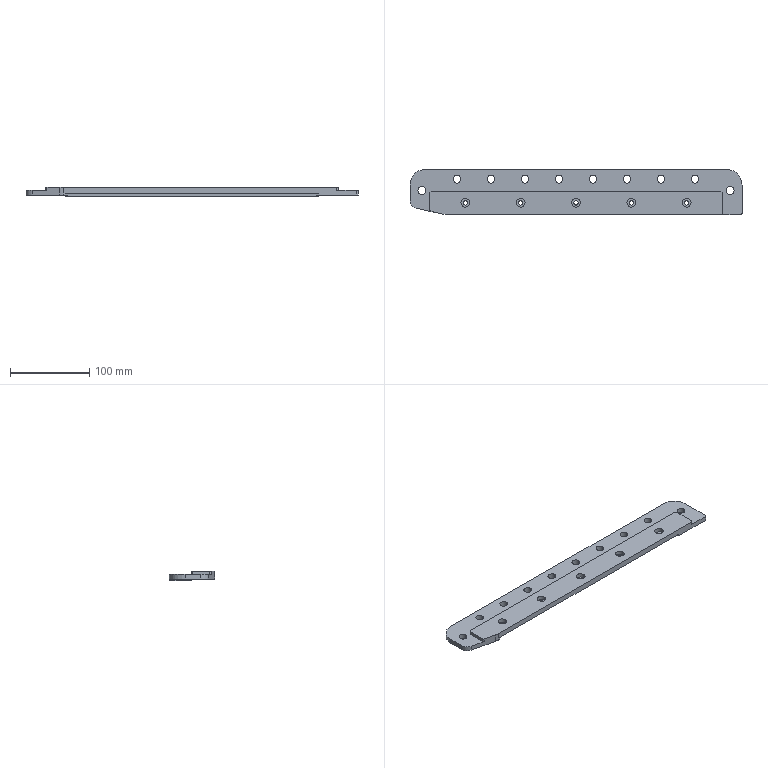Component | SolidWorks | 170423A4-PulleyRetainingPlate2-1 | 1 solid | 80 faces | box 420 x 57.5 x 12 mm | volume 171578 mm3 | cylinder 54 | plane 26 | commonest cylinder face diameters 10 x20 11 x10 5.5 x10 4 x7 2 x3 40 x3 20 x1
build123d program:
from build123d import *

# Parameters (mm, degrees)
SKETCH1_W                                       = 420
SKETCH1_H                                       = 57.5
BOSS_EXTRUDE1_DEPTH                             = 6
F_10_0_10_DIAMETER_HOLE1_D                      = 10
SKETCH4_W                                       = 320.2
SKETCH4_H                                       = 30
CUT_EXTRUDE1_DEPTH                              = 2.5
FILLET1_R                                       = 20
SKETCH9_W                                       = 320.2
SKETCH9_H                                       = 27.5
BOSS_EXTRUDE2_DEPTH                             = 2
F_10_0_10_DIAMETER_HOLE2_D                      = 10
SKETCH10_W                                      = 370
SKETCH10_H                                      = 30
BOSS_EXTRUDE3_DEPTH                             = 4
CHAMFER1_SIZE                                   = 10
CHAMFER1_SIZE2                                  = 45
FILLET2_R                                       = 10
FILLET3_R                                       = 20
FILLET4_R                                       = 2
CUT_EXTRUDE2_DEPTH                              = 2.5
CHAMFER2_SIZE                                   = 2
M5_HEX_SOCKET_HEAD_CAP_SCREW_CBORE1_D           = 5.5
M5_HEX_SOCKET_HEAD_CAP_SCREW_CBORE1_CBORE_D     = 11
M5_HEX_SOCKET_HEAD_CAP_SCREW_CBORE1_CBORE_DEPTH = 5


with BuildPart() as part:
    # Sketch1 → Boss-Extrude1 (new body)
    with BuildSketch(Plane.XY):
        with Locations((0, 28.75)):
            Rectangle(SKETCH1_W, SKETCH1_H)
    extrude(amount=BOSS_EXTRUDE1_DEPTH)

    # 10.0 _10_ Diameter Hole1 (through all)
    with Locations(Plane.XY.offset(6)):
        with Locations((-195, 30.5), (195, 30.5)):
            Hole(F_10_0_10_DIAMETER_HOLE1_D / 2)

    # Sketch4 → Cut-Extrude1 (cut)
    with BuildSketch(Plane(origin=(0, 0, 0), x_dir=(-1, 0, 0), z_dir=(0, 0, -1))):
        with Locations((0, 15)):
            Rectangle(SKETCH4_W, SKETCH4_H)
    extrude(amount=-CUT_EXTRUDE1_DEPTH, mode=Mode.SUBTRACT)

    # Fillet1
    fillet1_edges = [part.edges().sort_by_distance(p)[0] for p in [
        (-210, 57.5, 3),
        (210, 57.5, 3),
    ]]
    fillet(fillet1_edges, radius=FILLET1_R)

    # Sketch9 → Boss-Extrude2 (add)
    with BuildSketch(Plane(origin=(0, 0, 0), x_dir=(-1, 0, 0), z_dir=(0, 0, -1))):
        with Locations((0, 43.75)):
            Rectangle(SKETCH9_W, SKETCH9_H)
    extrude(amount=BOSS_EXTRUDE2_DEPTH)

    # 10.0 _10_ Diameter Hole2 (through all)
    with Locations(Plane.XY.offset(6)):
        with Locations((-150.5, 45), (-107.5, 45), (-64.5, 45), (-21.5, 45), (21.5, 45), (64.5, 45), (107.5, 45), (150.5, 45)):
            Hole(F_10_0_10_DIAMETER_HOLE2_D / 2)

    # Sketch10 → Boss-Extrude3 (add)
    with BuildSketch(Plane.XY.offset(6)):
        with Locations((0, 15)):
            Rectangle(SKETCH10_W, SKETCH10_H)
    extrude(amount=BOSS_EXTRUDE3_DEPTH)

    # Chamfer1
    chamfer1_edges = [part.edges().sort_by_distance(p)[0] for p in [
        (-210, 0, 3),
    ]]
    chamfer1_side = [part.faces().sort_by_distance(p)[0] for p in [
        (-210, 18.75, 3),
    ]]
    chamfer(chamfer1_edges, length=CHAMFER1_SIZE, length2=CHAMFER1_SIZE2, reference=chamfer1_side[0])

    # Fillet2
    fillet2_edges = [part.edges().sort_by_distance(p)[0] for p in [
        (-210, 10, 3),
    ]]
    fillet(fillet2_edges, radius=FILLET2_R)

    # Fillet3
    fillet3_edges = [part.edges().sort_by_distance(p)[0] for p in [
        (-165, 0, 5),
    ]]
    fillet(fillet3_edges, radius=FILLET3_R)

    # Fillet4
    fillet4_edges = [part.edges().sort_by_distance(p)[0] for p in [
        (185, 0, 8),
        (-185, 4.444, 8),
        (160.1, 57.5, -1),
        (160.1, 30, -1),
        (-160.1, 30, -1),
        (-160.1, 57.5, -1),
        (210, 0, 3),
    ]]
    fillet(fillet4_edges, radius=FILLET4_R)

    # Sketch11 → Cut-Extrude2 (cut)
    with BuildSketch(Plane(origin=(0, 0, 0), x_dir=(-1, 0, 0), z_dir=(0, 0, -1))):
        with BuildLine():
            Line((-160.1, 30), (160.1, 30))
            ThreePointArc((160.1, 30), (161.1, 29), (160.1, 28))
            Line((160.1, 28), (-160.1, 28))
            ThreePointArc((-160.1, 28), (-161.1, 29), (-160.1, 30))
        make_face()
    extrude(amount=-CUT_EXTRUDE2_DEPTH, mode=Mode.SUBTRACT)

    # Chamfer2
    chamfer2_edges = [part.edges().sort_by_distance(p)[0] for p in [
        (-185, 30, 8),
        (185, 30, 8),
    ]]
    chamfer(chamfer2_edges, length=CHAMFER2_SIZE)

    # M5 Hex Socket Head Cap Screw CBORE1 (through all)
    with Locations(Plane.XY.offset(10)):
        with Locations((-140, 15), (-70, 15), (70, 15), (140, 15), (0, 15)):
            CounterBoreHole(M5_HEX_SOCKET_HEAD_CAP_SCREW_CBORE1_D / 2, M5_HEX_SOCKET_HEAD_CAP_SCREW_CBORE1_CBORE_D / 2, M5_HEX_SOCKET_HEAD_CAP_SCREW_CBORE1_CBORE_DEPTH)


solid = part.part

# Placed as in the assembly
solid = solid.moved(Location((-55.246, -36.288, 461), (0, 0, 0)))